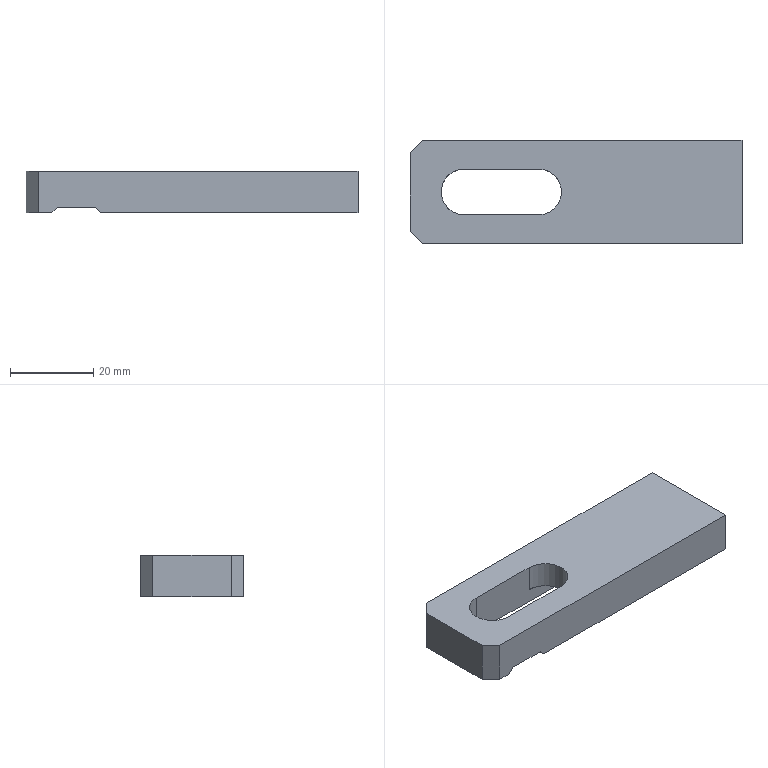Component | NX | CLAMP_PLATE_2 | 1 solid | 20 faces | volume 15051 mm3 | plane 18 | cylinder 2 | commonest cylinder face diameters 11 x2